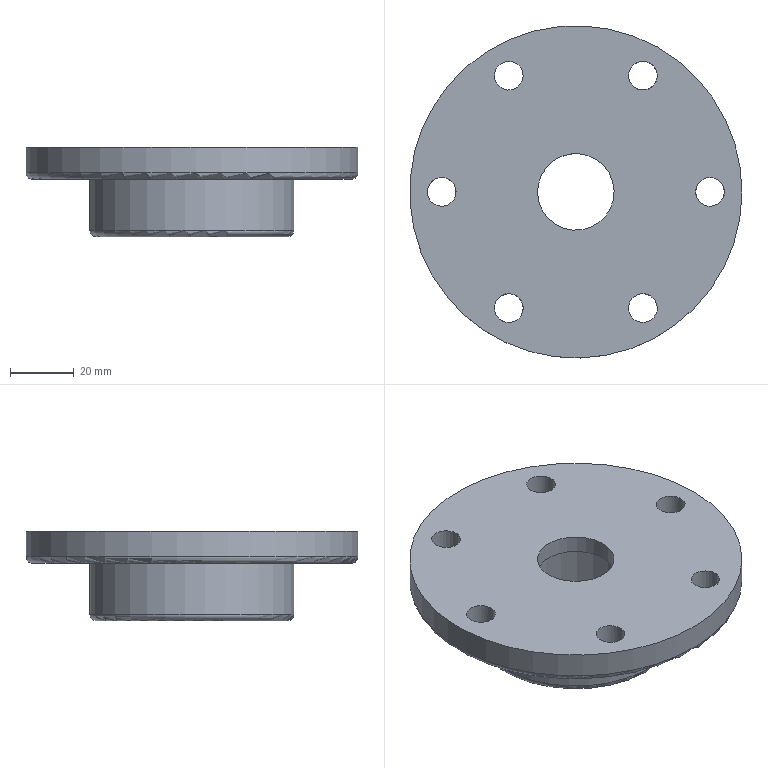Component | NX | END_CAP | 1 solid | 19 faces | volume 104184 mm3 | cylinder 11 | plane 5 | torus 2 | cone 1 | commonest cylinder face diameters 9 x6 104 x1 64 x1 42 x1 24 x1 44 x1